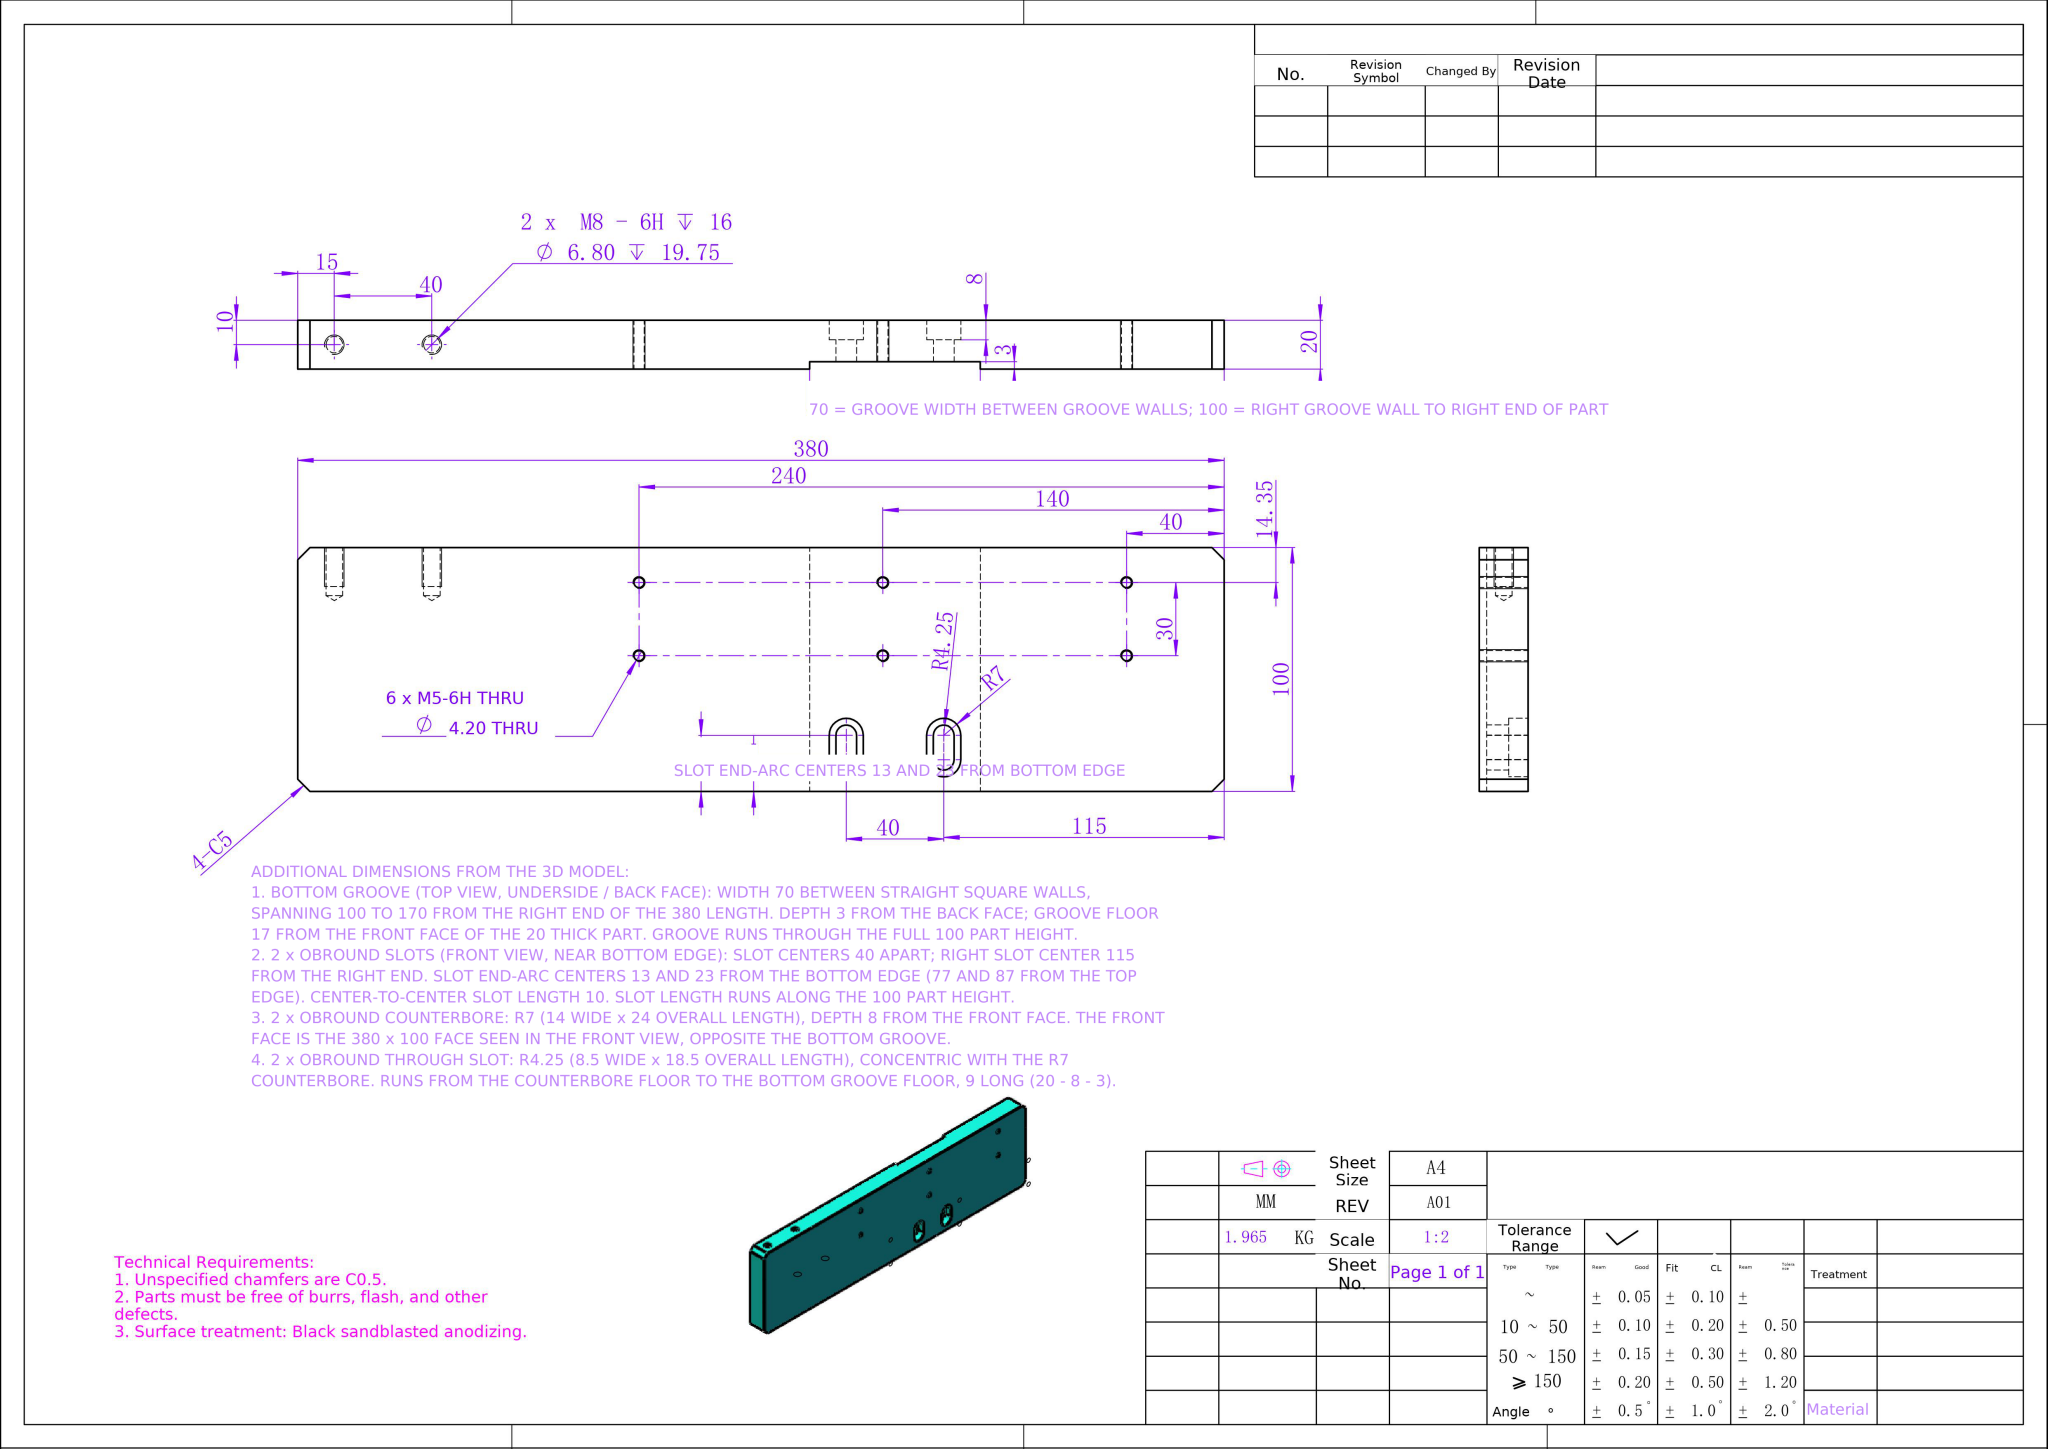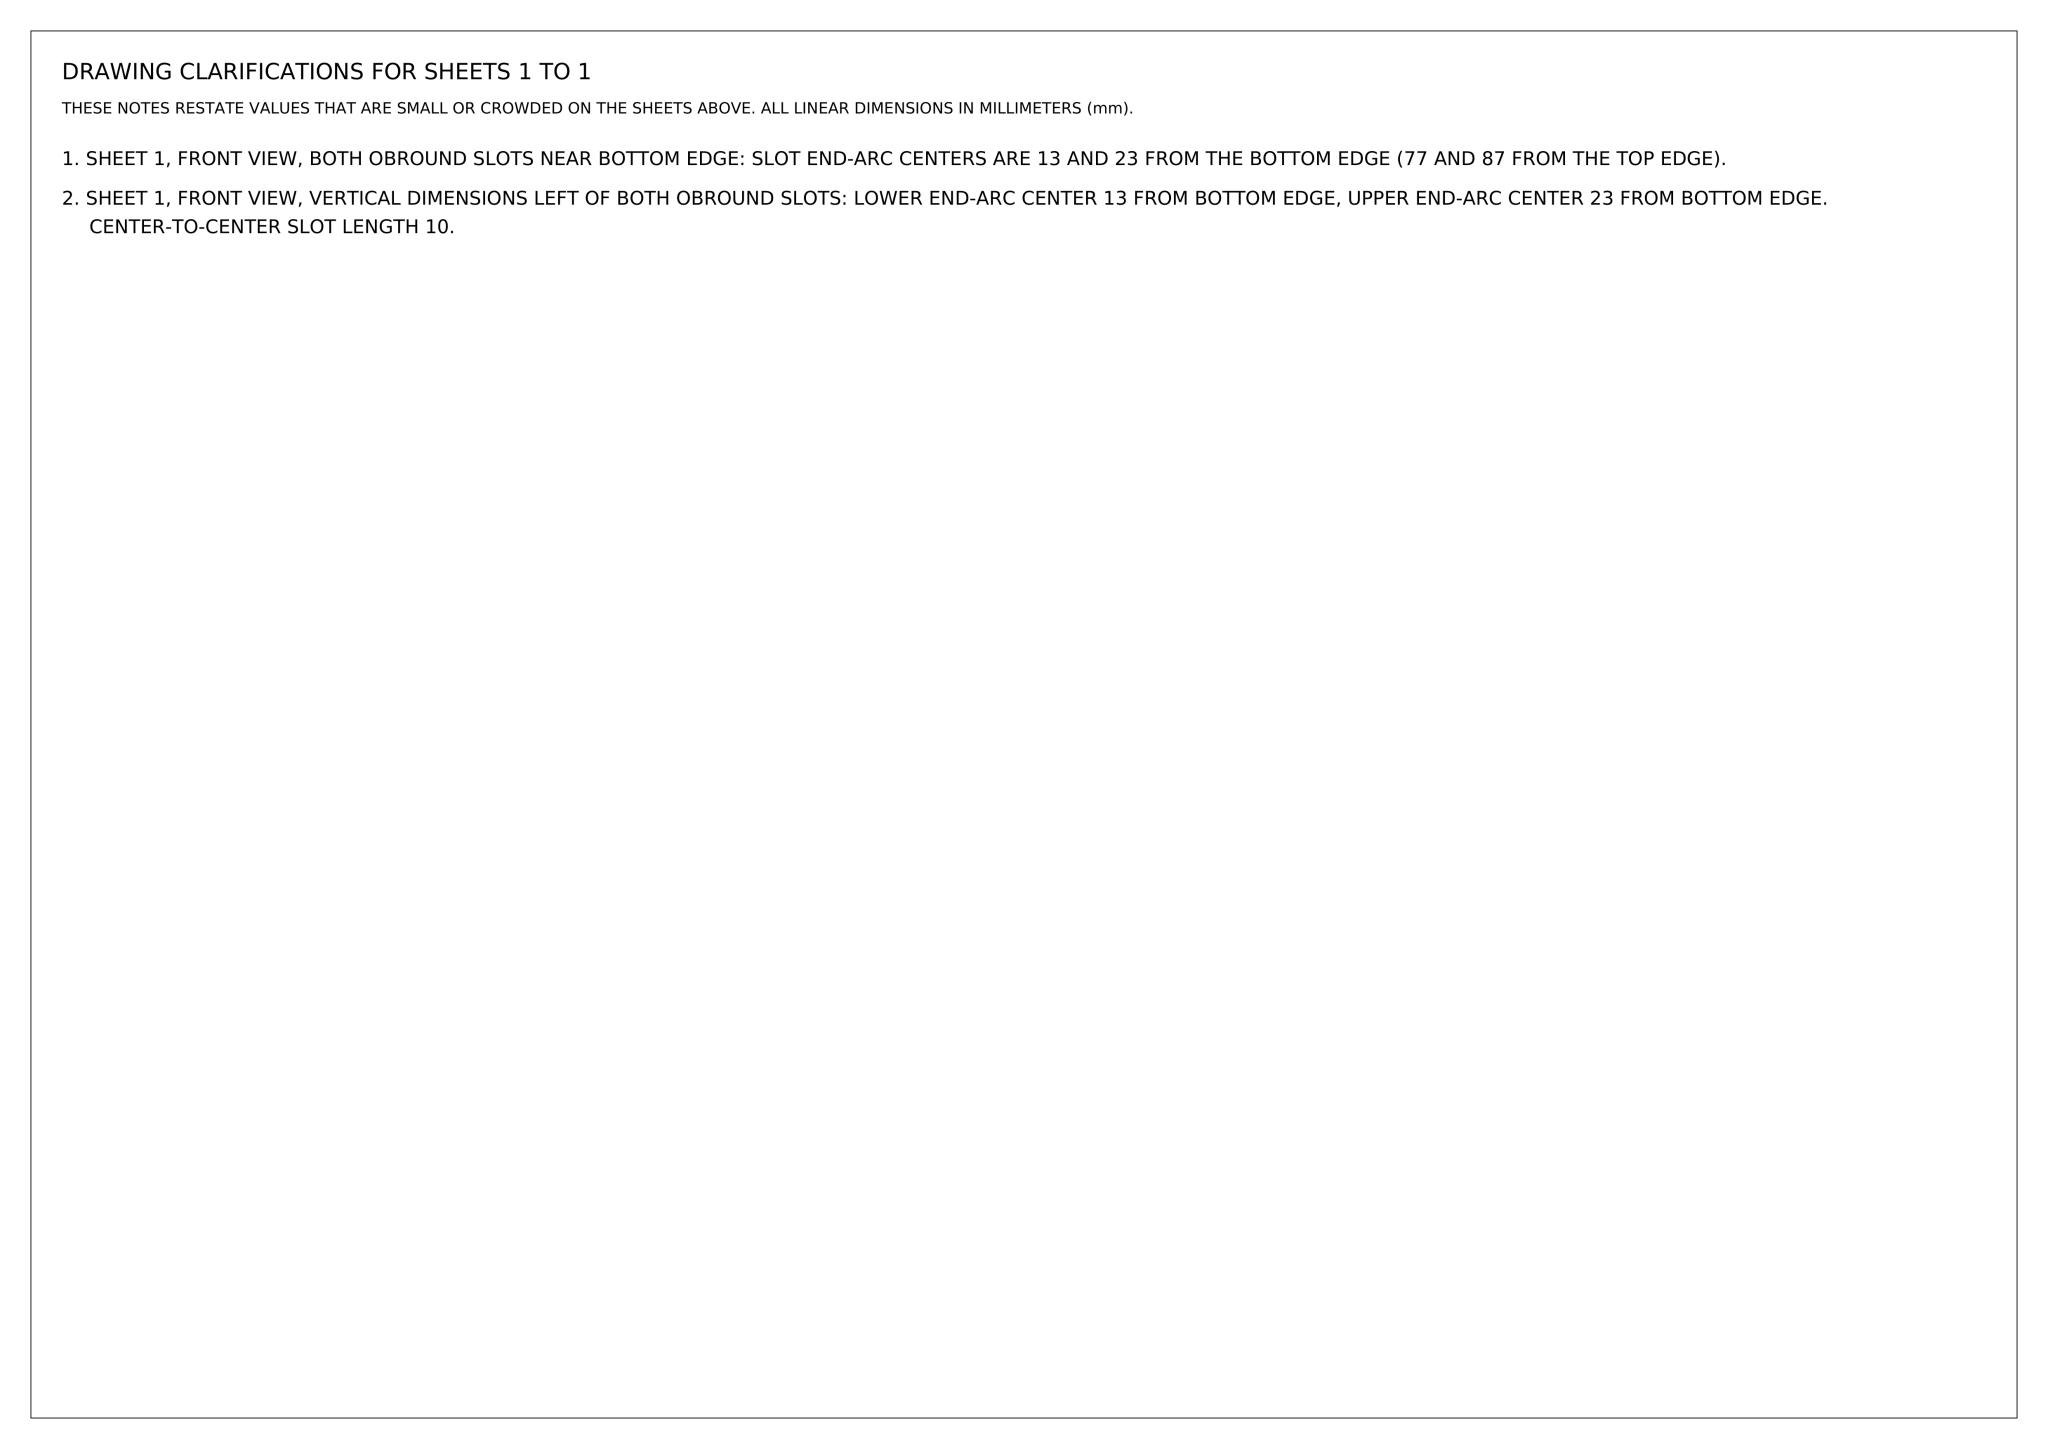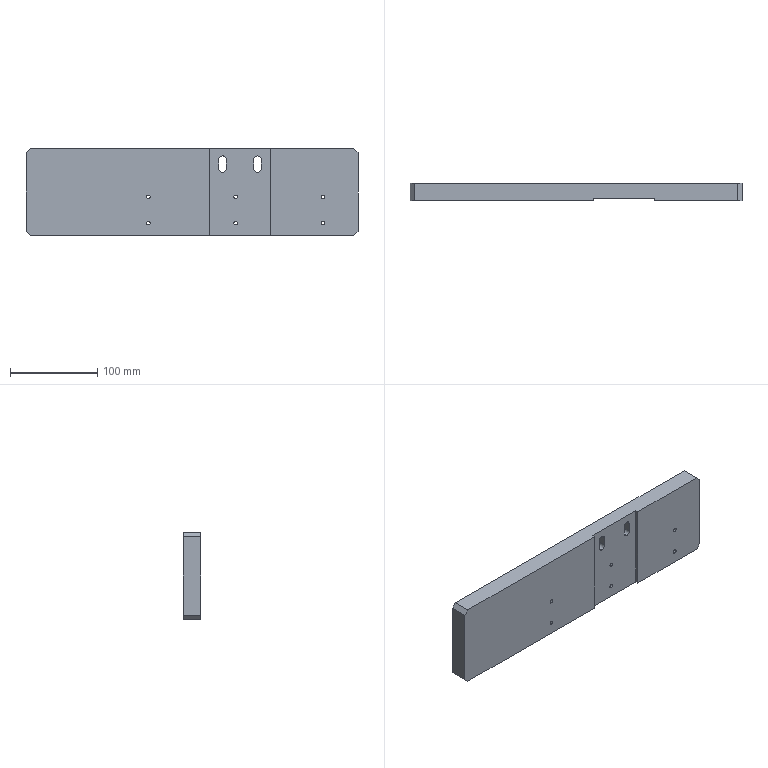Part | NX | mm | 1 solid | 56 faces | box 380 x 20 x 100 mm | volume 727682 mm3 | cylinder 28 | plane 24 | cone 4 | commonest cylinder face diameters 4.2 x12 14 x6 8.5 x6 6.8 x4